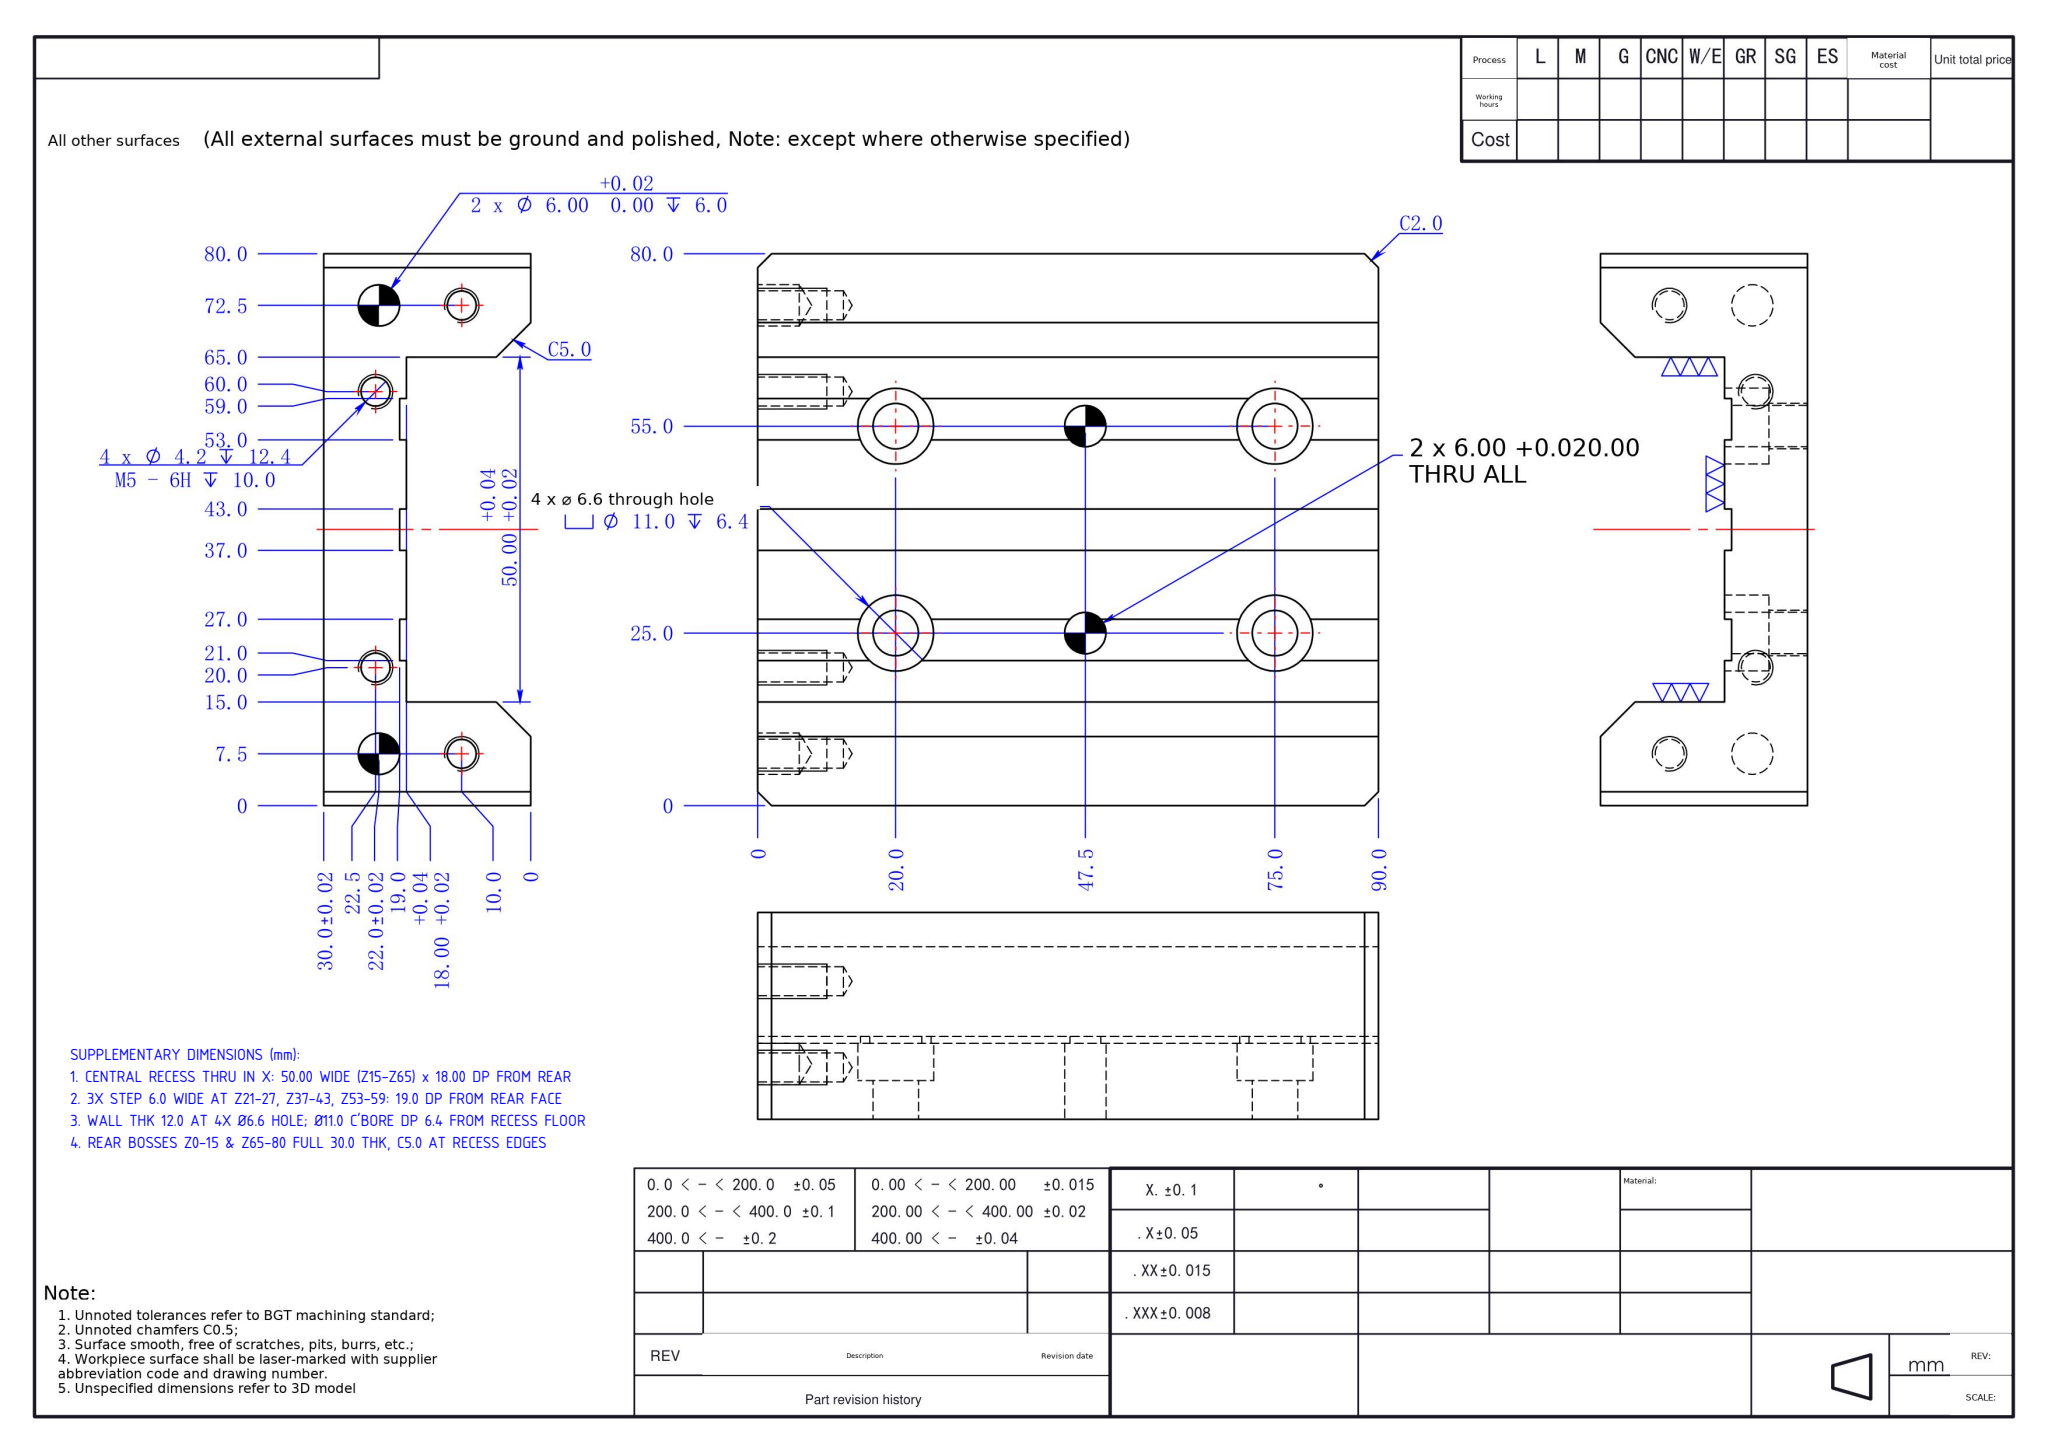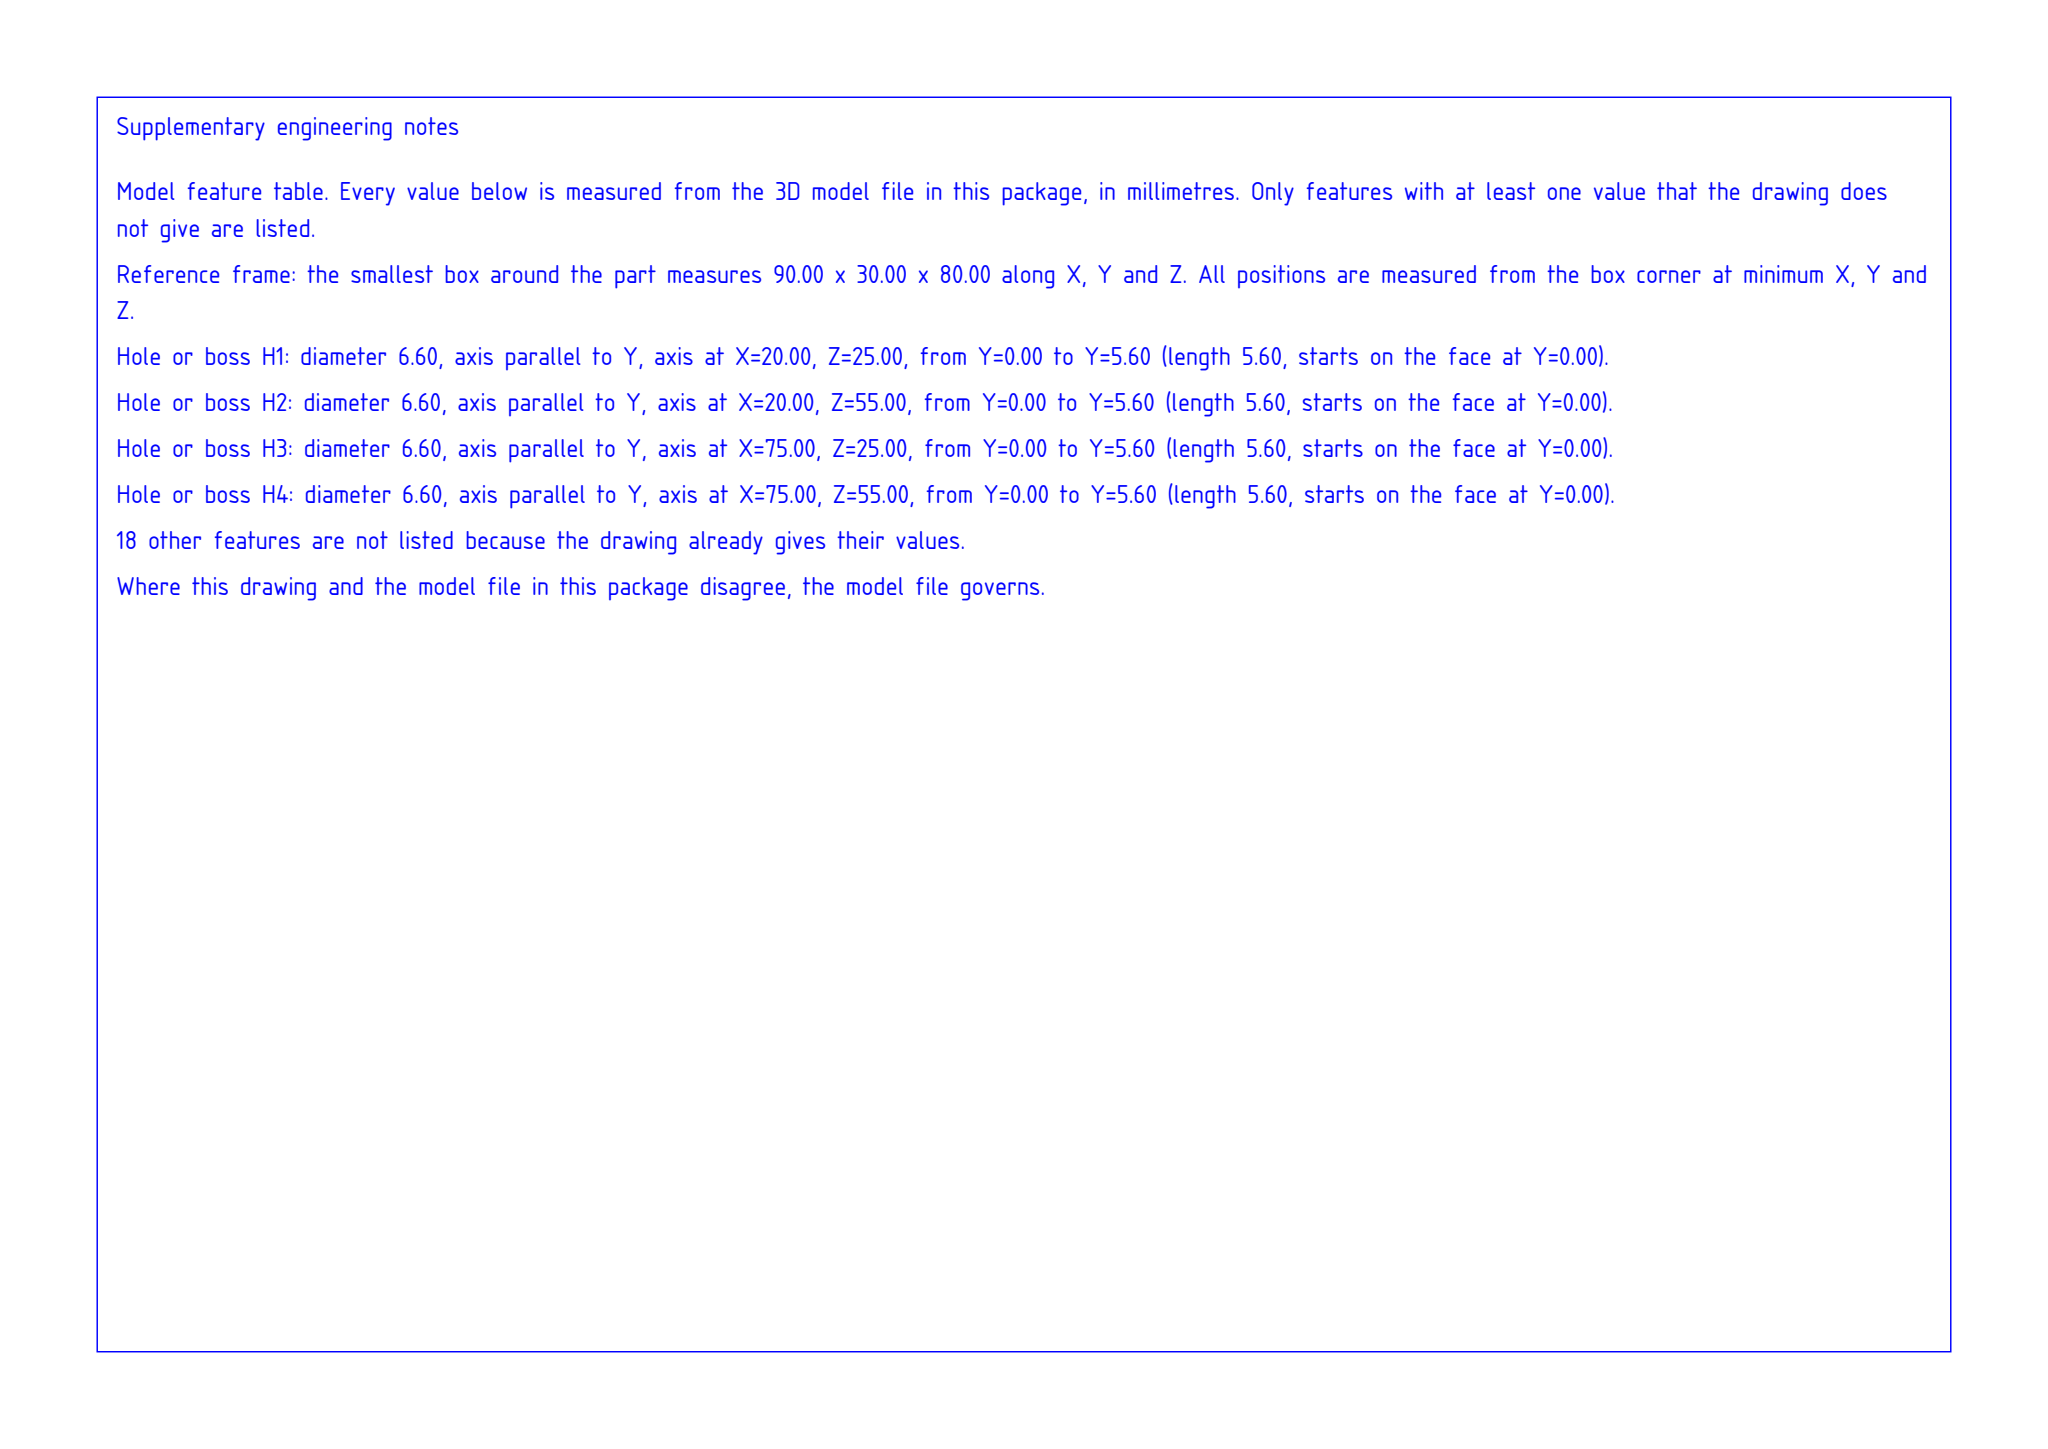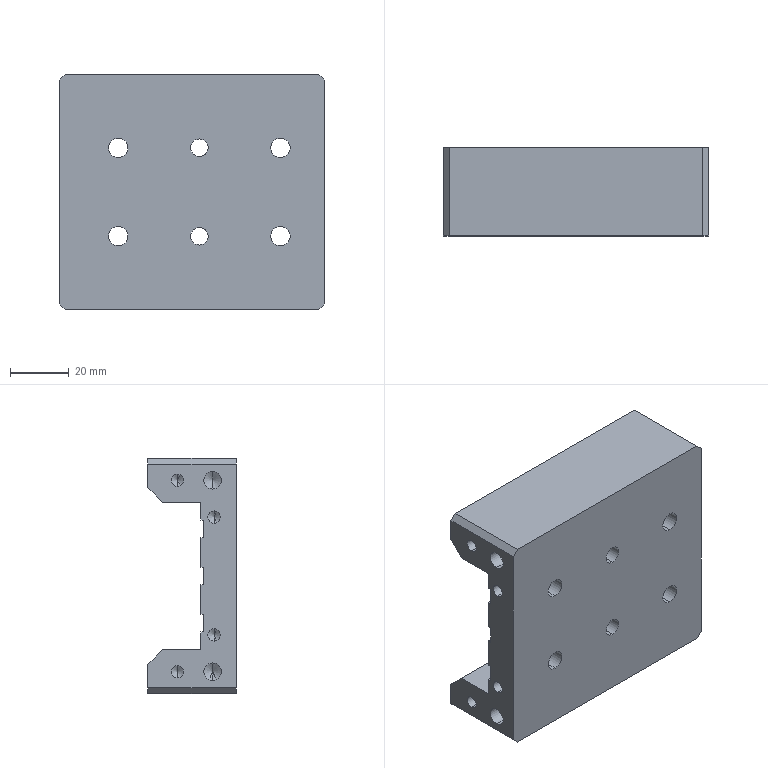Part | SolidWorks | mm | 1 solid | 90 faces | box 90 x 30 x 80 mm | volume 126224 mm3 | plane 46 | cylinder 32 | cone 12 | commonest cylinder face diameters 6 x8 4.2 x8 11 x8 6.6 x8
build123d program:
from build123d import *

# Parameters (mm, degrees)
SKETCH1_W                                       = 90
SKETCH1_H                                       = 80
BOSS_EXTRUDE1_DEPTH                             = 30
SKETCH2_W                                       = 90
SKETCH2_H                                       = 50
CUT_EXTRUDE1_DEPTH                              = 18
M6_HEX_SOCKET_HEAD_CAP_SCREW_CBORE1_D           = 6.6
M6_HEX_SOCKET_HEAD_CAP_SCREW_CBORE1_CBORE_D     = 11
M6_HEX_SOCKET_HEAD_CAP_SCREW_CBORE1_CBORE_DEPTH = 6.4
SIZE_MM_DOWEL_PIN_HOLE1_D                       = 6
CHAMFER1_SIZE                                   = 2
CHAMFER2_SIZE                                   = 5
M5_TAPPED_HOLE1_D                               = 4.2
M5_TAPPED_HOLE1_DEPTH                           = 12.4
M5_TAPPED_HOLE1_TIP                             = 1.262
SIZE_MM_DOWEL_PIN_HOLE2_D                       = 6
SIZE_MM_DOWEL_PIN_HOLE2_DEPTH                   = 6
SIZE_MM_DOWEL_PIN_HOLE2_TIP                     = 1.803
SKETCH11_W                                      = 6
SKETCH11_H                                      = 1
CUT_EXTRUDE2_DEPTH                              = 125.097


with BuildPart() as part:
    # Sketch1 → Boss-Extrude1 (new body)
    with BuildSketch(Plane(origin=(0, 0, 0), x_dir=(1, 0, 0), z_dir=(0, 1, 0))):
        with Locations((45, 40)):
            Rectangle(SKETCH1_W, SKETCH1_H)
    extrude(amount=BOSS_EXTRUDE1_DEPTH)

    # Sketch2 → Cut-Extrude1 (cut)
    with BuildSketch(Plane(origin=(0, 30, 0), x_dir=(1, 0, 0), z_dir=(0, 1, 0))):
        with Locations((45, 40)):
            Rectangle(SKETCH2_W, SKETCH2_H)
    extrude(amount=-CUT_EXTRUDE1_DEPTH, mode=Mode.SUBTRACT)

    # M6 Hex Socket Head Cap Screw CBORE1 (through all)
    with Locations(Plane(origin=(0, 12, 0), x_dir=(1, 0, 0), z_dir=(0, 1, 0))):
        with Locations((20, 25), (75, 25), (20, 55), (75, 55)):
            CounterBoreHole(M6_HEX_SOCKET_HEAD_CAP_SCREW_CBORE1_D / 2, M6_HEX_SOCKET_HEAD_CAP_SCREW_CBORE1_CBORE_D / 2, M6_HEX_SOCKET_HEAD_CAP_SCREW_CBORE1_CBORE_DEPTH)

    # Size mm Dowel Pin Hole1 (through all)
    with Locations(Plane(origin=(0, 30, 0), x_dir=(1, 0, 0), z_dir=(0, 1, 0))):
        with Locations((47.5, 55), (47.5, 25)):
            Hole(SIZE_MM_DOWEL_PIN_HOLE1_D / 2)

    # Chamfer1
    chamfer1_edges = [part.edges().sort_by_distance(p)[0] for p in [
        (0, 15, -80),
        (90, 15, -80),
        (90, 15, 0),
        (0, 15, 0),
    ]]
    chamfer(chamfer1_edges, length=CHAMFER1_SIZE)

    # Chamfer2
    chamfer2_edges = [part.edges().sort_by_distance(p)[0] for p in [
        (45, 30, -15),
        (45, 30, -65),
    ]]
    chamfer(chamfer2_edges, length=CHAMFER2_SIZE)

    # M5 Tapped Hole1
    with Locations(Plane.ZY):
        with Locations((-7.5, 20), (-20, 7.5), (-60, 7.5), (-72.5, 20)):
            Hole(M5_TAPPED_HOLE1_D / 2, depth=M5_TAPPED_HOLE1_DEPTH)
            with Locations((0, 0, -(M5_TAPPED_HOLE1_DEPTH + M5_TAPPED_HOLE1_TIP / 2))):  # 118° drill point
                Cone(0, M5_TAPPED_HOLE1_D / 2, M5_TAPPED_HOLE1_TIP, mode=Mode.SUBTRACT)

    # Size mm Dowel Pin Hole2
    with Locations(Plane.ZY):
        with Locations((-7.5, 8), (-72.5, 8)):
            Hole(SIZE_MM_DOWEL_PIN_HOLE2_D / 2, depth=SIZE_MM_DOWEL_PIN_HOLE2_DEPTH)
            with Locations((0, 0, -(SIZE_MM_DOWEL_PIN_HOLE2_DEPTH + SIZE_MM_DOWEL_PIN_HOLE2_TIP / 2))):  # 118° drill point
                Cone(0, SIZE_MM_DOWEL_PIN_HOLE2_D / 2, SIZE_MM_DOWEL_PIN_HOLE2_TIP, mode=Mode.SUBTRACT)

    # Sketch11 → Cut-Extrude2 (cut, through all)
    with BuildSketch(Plane(origin=(90, 0, 0), x_dir=(0, 0, -1), z_dir=(1, 0, 0))):
        with Locations((40, 11.5)):
            Rectangle(SKETCH11_W, SKETCH11_H)
        with Locations((24, 11.5)):
            Rectangle(SKETCH11_W, SKETCH11_H)
        with Locations((56, 11.5)):
            Rectangle(SKETCH11_W, SKETCH11_H)
    extrude(amount=-CUT_EXTRUDE2_DEPTH, mode=Mode.SUBTRACT)


solid = part.part